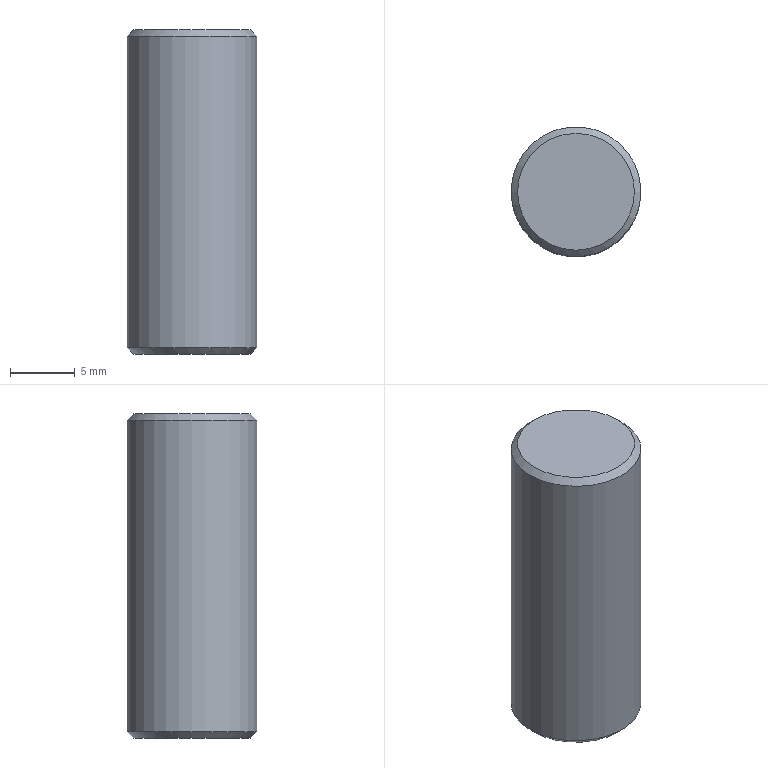Component | NX | PIN_2 | 1 solid | 5 faces | volume 1956 mm3 | plane 2 | cone 2 | cylinder 1 | commonest cylinder face diameters 10 x1